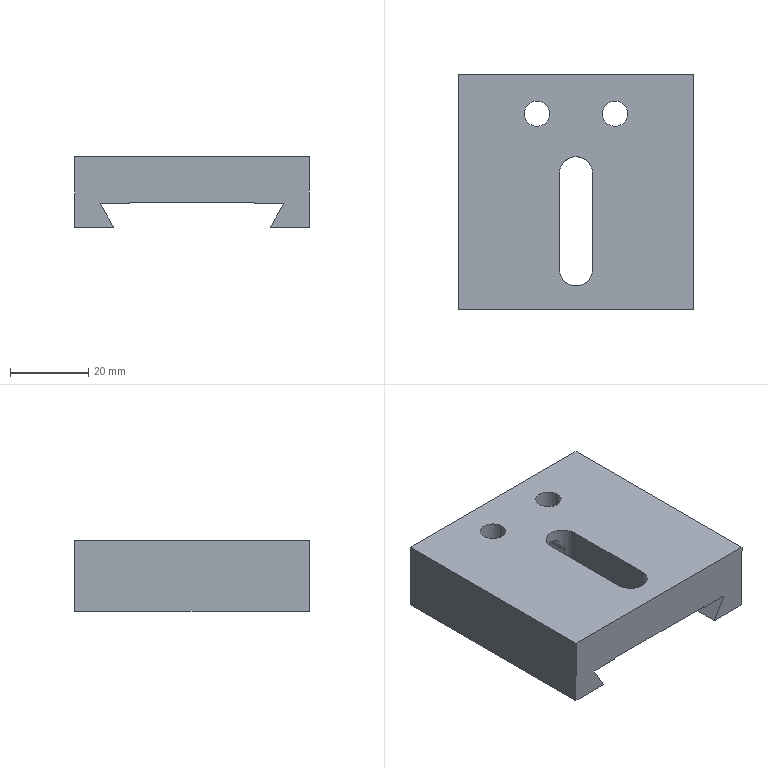Component | SolidWorks | DovetailBase2-1 | 1 solid | 30 faces | box 60 x 60 x 18 mm | volume 43120 mm3 | plane 18 | cylinder 12 | commonest cylinder face diameters 11 x4 6.5 x4 6.8 x2 8.5 x2
build123d program:
from build123d import *

# Parameters (mm, degrees)
SKETCH1_W                                          = 60
SKETCH1_H                                          = 60
BOSS_EXTRUDE1_DEPTH                                = 18
CUT_EXTRUDE1_DEPTH                                 = 72
SKETCH3_W                                          = 32
SKETCH3_H                                          = 60
CUT_EXTRUDE2_DEPTH                                 = 0.3
HOLE_SIZE_ACCORDING_TO_TYPE_1_OF_HEXAG_D           = 6.5
HOLE_SIZE_ACCORDING_TO_TYPE_1_OF_HEXAG_DEPTH       = 12.4
HOLE_SIZE_ACCORDING_TO_TYPE_1_OF_HEXAG_CBORE_D     = 11
HOLE_SIZE_ACCORDING_TO_TYPE_1_OF_HEXAG_CBORE_DEPTH = 6.5
HOLE_SIZE_ACCORDING_TO_TYPE_1_OF_HEXAG_TIP         = 1.953
CUT_EXTRUDE3_DEPTH                                 = 90.3
M8_TAPPED_HOLE1_REACH                              = 70.147
M8_TAPPED_HOLE1_BORE_R                             = 3.4


with BuildPart() as part:
    # Sketch1 → Boss-Extrude1 (new body)
    with BuildSketch(Plane.XY):
        Rectangle(SKETCH1_W, SKETCH1_H)
    extrude(amount=BOSS_EXTRUDE1_DEPTH)

    # Sketch2 → Cut-Extrude1 (cut)
    with BuildSketch(Plane(origin=(0, 30, 0), x_dir=(1, 0, 0), z_dir=(0, 1, 0))):
        Polygon((-20, -18), (-23.464, -12), (23.464, -12), (20, -18), align=None)
    extrude(amount=-CUT_EXTRUDE1_DEPTH, mode=Mode.SUBTRACT)

    # Sketch3 → Cut-Extrude2 (cut)
    with BuildSketch(Plane.XY.offset(12)):
        Rectangle(SKETCH3_W, SKETCH3_H)
    extrude(amount=-CUT_EXTRUDE2_DEPTH, mode=Mode.SUBTRACT)

    # Hole Size _according to_ Type 1 of Hexag
    with Locations(Plane(origin=(-10, 20, 11.7), x_dir=(1, 0, 0), z_dir=(0, 0, 1))):
        with Locations((0, 0), (20, 0)):
            CounterBoreHole(HOLE_SIZE_ACCORDING_TO_TYPE_1_OF_HEXAG_D / 2, HOLE_SIZE_ACCORDING_TO_TYPE_1_OF_HEXAG_CBORE_D / 2, HOLE_SIZE_ACCORDING_TO_TYPE_1_OF_HEXAG_CBORE_DEPTH, depth=HOLE_SIZE_ACCORDING_TO_TYPE_1_OF_HEXAG_DEPTH)
            with Locations((0, 0, -(HOLE_SIZE_ACCORDING_TO_TYPE_1_OF_HEXAG_DEPTH + HOLE_SIZE_ACCORDING_TO_TYPE_1_OF_HEXAG_TIP / 2))):  # 118° drill point
                Cone(0, HOLE_SIZE_ACCORDING_TO_TYPE_1_OF_HEXAG_D / 2, HOLE_SIZE_ACCORDING_TO_TYPE_1_OF_HEXAG_TIP, mode=Mode.SUBTRACT)

    # Sketch5 → Cut-Extrude3 (cut)
    with BuildSketch(Plane.XY.offset(11.7)):
        with BuildLine():
            Line((-4.25, -19.75), (-4.25, 4.75))
            ThreePointArc((-4.25, 4.75), (0, 9), (4.25, 4.75))
            Line((4.25, 4.75), (4.25, -19.75))
            ThreePointArc((4.25, -19.75), (0, -24), (-4.25, -19.75))
        make_face()
    extrude(amount=-CUT_EXTRUDE3_DEPTH, mode=Mode.SUBTRACT)

    # M8 Tapped Hole1 bore (on position points) → M8 Tapped Hole1 (cut, up to next)
    with BuildSketch(Plane(origin=(0, 30, 6), x_dir=(0, 0, 1), z_dir=(0, 1, 0)), mode=Mode.PRIVATE) as m8_tapped_hole1_sk1:
        Circle(M8_TAPPED_HOLE1_BORE_R)
    m8_tapped_hole1_tool1 = extrude(m8_tapped_hole1_sk1.sketch, amount=-M8_TAPPED_HOLE1_REACH, mode=Mode.PRIVATE) & part.part
    add(m8_tapped_hole1_tool1.solids().sort_by_distance((0, 30, 6))[0], mode=Mode.SUBTRACT)


solid = part.part

# Placed as in the assembly
solid = solid.moved(Location((-48.047, -14.04, 21), (-180, 0, 180)))
STEP:
#1=CARTESIAN_POINT('',(-1.892,-0.1984,0.7244));
#2=VERTEX_POINT('',#1);
#3=CARTESIAN_POINT('',(-1.892,-0.1984,0.4567));
#4=VERTEX_POINT('',#3);
#5=CARTESIAN_POINT('',(-1.892,-0.1984,0.7244));
#6=CARTESIAN_POINT('',(-1.882,-0.1984,0.7244));
#7=CARTESIAN_POINT('',(-1.873,-0.1992,0.7234));
#8=CARTESIAN_POINT('',(-1.855,-0.2022,0.7197));
#9=CARTESIAN_POINT('',(-1.846,-0.2044,0.7169));
#10=CARTESIAN_POINT('',(-1.83,-0.2099,0.7098));
#11=CARTESIAN_POINT('',(-1.823,-0.2131,0.7056));
#12=CARTESIAN_POINT('',(-1.808,-0.2203,0.6958));
#13=CARTESIAN_POINT('',(-1.802,-0.2243,0.6903));
#14=CARTESIAN_POINT('',(-1.79,-0.2324,0.6785));
#15=CARTESIAN_POINT('',(-1.785,-0.2366,0.672));
#16=CARTESIAN_POINT('',(-1.776,-0.2448,0.6582));
#17=CARTESIAN_POINT('',(-1.772,-0.2488,0.6509));
#18=CARTESIAN_POINT('',(-1.767,-0.2542,0.6392));
#19=CARTESIAN_POINT('',(-1.765,-0.2559,0.6352));
#20=CARTESIAN_POINT('',(-1.763,-0.259,0.6269));
#21=CARTESIAN_POINT('',(-1.762,-0.2605,0.6225));
#22=CARTESIAN_POINT('',(-1.76,-0.2628,0.6137));
#23=CARTESIAN_POINT('',(-1.759,-0.2637,0.6092));
#24=CARTESIAN_POINT('',(-1.758,-0.265,0.6));
#25=CARTESIAN_POINT('',(-1.758,-0.2653,0.5953));
#26=CARTESIAN_POINT('',(-1.758,-0.2654,0.5813));
#27=CARTESIAN_POINT('',(-1.759,-0.264,0.5721));
#28=CARTESIAN_POINT('',(-1.762,-0.2594,0.5544));
#29=CARTESIAN_POINT('',(-1.765,-0.2562,0.5461));
#30=CARTESIAN_POINT('',(-1.772,-0.2489,0.5303));
#31=CARTESIAN_POINT('',(-1.776,-0.2448,0.5229));
#32=CARTESIAN_POINT('',(-1.785,-0.2366,0.5092));
#33=CARTESIAN_POINT('',(-1.79,-0.2324,0.5027));
#34=CARTESIAN_POINT('',(-1.802,-0.2243,0.4908));
#35=CARTESIAN_POINT('',(-1.808,-0.2203,0.4853));
#36=CARTESIAN_POINT('',(-1.822,-0.2132,0.4757));
#37=CARTESIAN_POINT('',(-1.83,-0.21,0.4714));
#38=CARTESIAN_POINT('',(-1.846,-0.2045,0.4643));
#39=CARTESIAN_POINT('',(-1.855,-0.2022,0.4615));
#40=CARTESIAN_POINT('',(-1.873,-0.1992,0.4577));
#41=CARTESIAN_POINT('',(-1.882,-0.1984,0.4567));
#42=CARTESIAN_POINT('',(-1.892,-0.1984,0.4567));
#43=B_SPLINE_CURVE_WITH_KNOTS('',3,(#5,#6,#7,#8,#9,#10,#11,#12,#13,#14,#15,#16,#17,#18,#19,#20,#21,#22,#23,#24,#25,#26,#27,#28,#29,#30,#31,#32,#33,#34,#35,#36,#37,#38,#39,#40,#41,#42),.UNSPECIFIED.,.F.,.F.,(4,2,2,2,2,2,2,2,2,2,2,2,2,2,2,2,2,2,4),(0.01126,0.01196,0.01266,0.01336,0.01406,0.01477,0.01547,0.01582,0.01617,0.01652,0.01687,0.01757,0.01827,0.01897,0.01968,0.02038,0.02108,0.02178,0.02248),.UNSPECIFIED.);
#44=EDGE_CURVE('',#2,#4,#43,.T.);
#45=ORIENTED_EDGE('',*,*,#44,.F.);
#46=CARTESIAN_POINT('',(-1.892,0.6284,0.7244));
#47=VERTEX_POINT('',#46);
#48=CARTESIAN_POINT('',(-1.892,0.6284,0.7244));
#49=DIRECTION('',(-0.,1.,0.));
#50=VECTOR('',#49,39.37);
#51=LINE('',#48,#50);
#52=EDGE_CURVE('',#2,#47,#51,.T.);
#53=ORIENTED_EDGE('',*,*,#52,.T.);
#54=CARTESIAN_POINT('',(-1.892,0.6284,0.4567));
#55=VERTEX_POINT('',#54);
#56=CARTESIAN_POINT('',(-1.892,0.6284,0.5906));
#57=DIRECTION('',(-0.,1.,0.));
#58=DIRECTION('',(-0.,0.,-1.));
#59=AXIS2_PLACEMENT_3D('',#56,#57,#58);
#60=CIRCLE('',#59,0.1339);
#61=EDGE_CURVE('',#47,#55,#60,.T.);
#62=ORIENTED_EDGE('',*,*,#61,.T.);
#63=CARTESIAN_POINT('',(-1.892,0.6284,0.4567));
#64=DIRECTION('',(-0.,1.,0.));
#65=VECTOR('',#64,39.37);
#66=LINE('',#63,#65);
#67=EDGE_CURVE('',#4,#55,#66,.T.);
#68=ORIENTED_EDGE('',*,*,#67,.F.);
#69=EDGE_LOOP('',(#45,#53,#62,#68));
#70=FACE_OUTER_BOUND('',#69,.T.);
#71=CARTESIAN_POINT('',(-1.892,0.6284,0.5906));
#72=DIRECTION('',(-0.,1.,0.));
#73=DIRECTION('',(-0.,0.,-1.));
#74=AXIS2_PLACEMENT_3D('',#71,#72,#73);
#75=CYLINDRICAL_SURFACE('',#74,0.1339);
#76=ADVANCED_FACE('',(#70),#75,.F.);
#77=CARTESIAN_POINT('',(-1.281,0.2347,0.622));
#78=VERTEX_POINT('',#77);
#79=CARTESIAN_POINT('',(-1.714,0.2347,0.622));
#80=VERTEX_POINT('',#79);
#81=CARTESIAN_POINT('',(-1.498,0.2347,0.622));
#82=DIRECTION('',(-0.,0.,-1.));
#83=DIRECTION('',(-1.,0.,0.));
#84=AXIS2_PLACEMENT_3D('',#81,#82,#83);
#85=CIRCLE('',#84,0.2165);
#86=EDGE_CURVE('',#78,#80,#85,.T.);
#87=ORIENTED_EDGE('',*,*,#86,.F.);
#88=CARTESIAN_POINT('',(-1.281,0.2347,0.3661));
#89=VERTEX_POINT('',#88);
#90=CARTESIAN_POINT('',(-1.281,0.2347,0.3661));
#91=DIRECTION('',(-0.,0.,-1.));
#92=VECTOR('',#91,39.37);
#93=LINE('',#90,#92);
#94=EDGE_CURVE('',#78,#89,#93,.T.);
#95=ORIENTED_EDGE('',*,*,#94,.T.);
#96=CARTESIAN_POINT('',(-1.714,0.2347,0.3661));
#97=VERTEX_POINT('',#96);
#98=CARTESIAN_POINT('',(-1.498,0.2347,0.3661));
#99=DIRECTION('',(-0.,0.,-1.));
#100=DIRECTION('',(-1.,0.,0.));
#101=AXIS2_PLACEMENT_3D('',#98,#99,#100);
#102=CIRCLE('',#101,0.2165);
#103=EDGE_CURVE('',#89,#97,#102,.T.);
#104=ORIENTED_EDGE('',*,*,#103,.T.);
#105=CARTESIAN_POINT('',(-1.714,0.2347,0.3661));
#106=DIRECTION('',(-0.,0.,-1.));
#107=VECTOR('',#106,39.37);
#108=LINE('',#105,#107);
#109=EDGE_CURVE('',#80,#97,#108,.T.);
#110=ORIENTED_EDGE('',*,*,#109,.F.);
#111=EDGE_LOOP('',(#87,#95,#104,#110));
#112=FACE_OUTER_BOUND('',#111,.T.);
#113=CARTESIAN_POINT('',(-1.498,0.2347,0.3661));
#114=DIRECTION('',(-0.,0.,-1.));
#115=DIRECTION('',(-1.,0.,0.));
#116=AXIS2_PLACEMENT_3D('',#113,#114,#115);
#117=CYLINDRICAL_SURFACE('',#116,0.2165);
#118=ADVANCED_FACE('',(#112),#117,.F.);
#119=CARTESIAN_POINT('',(-1.626,0.2347,0.8268));
#120=VERTEX_POINT('',#119);
#121=CARTESIAN_POINT('',(-1.37,0.2347,0.8268));
#122=VERTEX_POINT('',#121);
#123=CARTESIAN_POINT('',(-1.498,0.2347,0.8268));
#124=DIRECTION('',(0.,-0.,1.));
#125=DIRECTION('',(1.,0.,-0.));
#126=AXIS2_PLACEMENT_3D('',#123,#124,#125);
#127=CIRCLE('',#126,0.128);
#128=EDGE_CURVE('',#120,#122,#127,.T.);
#129=ORIENTED_EDGE('',*,*,#128,.T.);
#130=CARTESIAN_POINT('',(-1.37,0.2347,0.622));
#131=VERTEX_POINT('',#130);
#132=CARTESIAN_POINT('',(-1.37,0.2347,0.3661));
#133=DIRECTION('',(-0.,0.,-1.));
#134=VECTOR('',#133,39.37);
#135=LINE('',#132,#134);
#136=EDGE_CURVE('',#122,#131,#135,.T.);
#137=ORIENTED_EDGE('',*,*,#136,.T.);
#138=CARTESIAN_POINT('',(-1.626,0.2347,0.622));
#139=VERTEX_POINT('',#138);
#140=CARTESIAN_POINT('',(-1.498,0.2347,0.622));
#141=DIRECTION('',(-0.,0.,-1.));
#142=DIRECTION('',(-1.,0.,0.));
#143=AXIS2_PLACEMENT_3D('',#140,#141,#142);
#144=CIRCLE('',#143,0.128);
#145=EDGE_CURVE('',#131,#139,#144,.T.);
#146=ORIENTED_EDGE('',*,*,#145,.T.);
#147=CARTESIAN_POINT('',(-1.626,0.2347,0.3661));
#148=DIRECTION('',(-0.,0.,-1.));
#149=VECTOR('',#148,39.37);
#150=LINE('',#147,#149);
#151=EDGE_CURVE('',#120,#139,#150,.T.);
#152=ORIENTED_EDGE('',*,*,#151,.F.);
#153=EDGE_LOOP('',(#129,#137,#146,#152));
#154=FACE_OUTER_BOUND('',#153,.T.);
#155=CARTESIAN_POINT('',(-1.498,0.2347,0.3661));
#156=DIRECTION('',(-0.,0.,-1.));
#157=DIRECTION('',(-1.,0.,0.));
#158=AXIS2_PLACEMENT_3D('',#155,#156,#157);
#159=CYLINDRICAL_SURFACE('',#158,0.128);
#160=ADVANCED_FACE('',(#154),#159,.F.);
#161=CARTESIAN_POINT('',(-2.069,0.2347,0.622));
#162=VERTEX_POINT('',#161);
#163=CARTESIAN_POINT('',(-2.502,0.2347,0.622));
#164=VERTEX_POINT('',#163);
#165=CARTESIAN_POINT('',(-2.285,0.2347,0.622));
#166=DIRECTION('',(-0.,0.,-1.));
#167=DIRECTION('',(-1.,0.,0.));
#168=AXIS2_PLACEMENT_3D('',#165,#166,#167);
#169=CIRCLE('',#168,0.2165);
#170=EDGE_CURVE('',#162,#164,#169,.T.);
#171=ORIENTED_EDGE('',*,*,#170,.F.);
#172=CARTESIAN_POINT('',(-2.069,0.2347,0.3661));
#173=VERTEX_POINT('',#172);
#174=CARTESIAN_POINT('',(-2.069,0.2347,0.3661));
#175=DIRECTION('',(-0.,0.,-1.));
#176=VECTOR('',#175,39.37);
#177=LINE('',#174,#176);
#178=EDGE_CURVE('',#162,#173,#177,.T.);
#179=ORIENTED_EDGE('',*,*,#178,.T.);
#180=CARTESIAN_POINT('',(-2.502,0.2347,0.3661));
#181=VERTEX_POINT('',#180);
#182=CARTESIAN_POINT('',(-2.285,0.2347,0.3661));
#183=DIRECTION('',(-0.,0.,-1.));
#184=DIRECTION('',(-1.,0.,0.));
#185=AXIS2_PLACEMENT_3D('',#182,#183,#184);
#186=CIRCLE('',#185,0.2165);
#187=EDGE_CURVE('',#173,#181,#186,.T.);
#188=ORIENTED_EDGE('',*,*,#187,.T.);
#189=CARTESIAN_POINT('',(-2.502,0.2347,0.3661));
#190=DIRECTION('',(-0.,0.,-1.));
#191=VECTOR('',#190,39.37);
#192=LINE('',#189,#191);
#193=EDGE_CURVE('',#164,#181,#192,.T.);
#194=ORIENTED_EDGE('',*,*,#193,.F.);
#195=EDGE_LOOP('',(#171,#179,#188,#194));
#196=FACE_OUTER_BOUND('',#195,.T.);
#197=CARTESIAN_POINT('',(-2.285,0.2347,0.3661));
#198=DIRECTION('',(-0.,0.,-1.));
#199=DIRECTION('',(-1.,0.,0.));
#200=AXIS2_PLACEMENT_3D('',#197,#198,#199);
#201=CYLINDRICAL_SURFACE('',#200,0.2165);
#202=ADVANCED_FACE('',(#196),#201,.F.);
#203=CARTESIAN_POINT('',(-2.413,0.2347,0.8268));
#204=VERTEX_POINT('',#203);
#205=CARTESIAN_POINT('',(-2.157,0.2347,0.8268));
#206=VERTEX_POINT('',#205);
#207=CARTESIAN_POINT('',(-2.285,0.2347,0.8268));
#208=DIRECTION('',(0.,-0.,1.));
#209=DIRECTION('',(1.,0.,-0.));
#210=AXIS2_PLACEMENT_3D('',#207,#208,#209);
#211=CIRCLE('',#210,0.128);
#212=EDGE_CURVE('',#204,#206,#211,.T.);
#213=ORIENTED_EDGE('',*,*,#212,.T.);
#214=CARTESIAN_POINT('',(-2.157,0.2347,0.622));
#215=VERTEX_POINT('',#214);
#216=CARTESIAN_POINT('',(-2.157,0.2347,0.3661));
#217=DIRECTION('',(-0.,0.,-1.));
#218=VECTOR('',#217,39.37);
#219=LINE('',#216,#218);
#220=EDGE_CURVE('',#206,#215,#219,.T.);
#221=ORIENTED_EDGE('',*,*,#220,.T.);
#222=CARTESIAN_POINT('',(-2.413,0.2347,0.622));
#223=VERTEX_POINT('',#222);
#224=CARTESIAN_POINT('',(-2.285,0.2347,0.622));
#225=DIRECTION('',(-0.,0.,-1.));
#226=DIRECTION('',(-1.,0.,0.));
#227=AXIS2_PLACEMENT_3D('',#224,#225,#226);
#228=CIRCLE('',#227,0.128);
#229=EDGE_CURVE('',#215,#223,#228,.T.);
#230=ORIENTED_EDGE('',*,*,#229,.T.);
#231=CARTESIAN_POINT('',(-2.413,0.2347,0.3661));
#232=DIRECTION('',(-0.,0.,-1.));
#233=VECTOR('',#232,39.37);
#234=LINE('',#231,#233);
#235=EDGE_CURVE('',#204,#223,#234,.T.);
#236=ORIENTED_EDGE('',*,*,#235,.F.);
#237=EDGE_LOOP('',(#213,#221,#230,#236));
#238=FACE_OUTER_BOUND('',#237,.T.);
#239=CARTESIAN_POINT('',(-2.285,0.2347,0.3661));
#240=DIRECTION('',(-0.,0.,-1.));
#241=DIRECTION('',(-1.,0.,0.));
#242=AXIS2_PLACEMENT_3D('',#239,#240,#241);
#243=CYLINDRICAL_SURFACE('',#242,0.128);
#244=ADVANCED_FACE('',(#238),#243,.F.);
#245=CARTESIAN_POINT('',(-2.815,0.6284,0.3543));
#246=VERTEX_POINT('',#245);
#247=CARTESIAN_POINT('',(-2.522,0.6284,0.3543));
#248=VERTEX_POINT('',#247);
#249=CARTESIAN_POINT('',(-0.9678,0.6284,0.3543));
#250=DIRECTION('',(1.,0.,-0.));
#251=VECTOR('',#250,39.37);
#252=LINE('',#249,#251);
#253=EDGE_CURVE('',#246,#248,#252,.T.);
#254=ORIENTED_EDGE('',*,*,#253,.T.);
#255=CARTESIAN_POINT('',(-2.522,-1.734,0.3543));
#256=VERTEX_POINT('',#255);
#257=CARTESIAN_POINT('',(-2.522,-1.734,0.3543));
#258=DIRECTION('',(-0.,1.,0.));
#259=VECTOR('',#258,39.37);
#260=LINE('',#257,#259);
#261=EDGE_CURVE('',#256,#248,#260,.T.);
#262=ORIENTED_EDGE('',*,*,#261,.F.);
#263=CARTESIAN_POINT('',(-2.815,-1.734,0.3543));
#264=VERTEX_POINT('',#263);
#265=CARTESIAN_POINT('',(-0.7105,-1.734,0.3543));
#266=DIRECTION('',(1.,0.,-0.));
#267=VECTOR('',#266,39.37);
#268=LINE('',#265,#267);
#269=EDGE_CURVE('',#264,#256,#268,.T.);
#270=ORIENTED_EDGE('',*,*,#269,.F.);
#271=CARTESIAN_POINT('',(-2.815,-2.206,0.3543));
#272=DIRECTION('',(-0.,1.,0.));
#273=VECTOR('',#272,39.37);
#274=LINE('',#271,#273);
#275=EDGE_CURVE('',#264,#246,#274,.T.);
#276=ORIENTED_EDGE('',*,*,#275,.T.);
#277=EDGE_LOOP('',(#254,#262,#270,#276));
#278=FACE_OUTER_BOUND('',#277,.T.);
#279=CARTESIAN_POINT('',(-0.9678,-2.206,0.3543));
#280=DIRECTION('',(0.,-0.,1.));
#281=DIRECTION('',(1.,0.,-0.));
#282=AXIS2_PLACEMENT_3D('',#279,#280,#281);
#283=PLANE('',#282);
#284=ADVANCED_FACE('',(#278),#283,.F.);
#285=CARTESIAN_POINT('',(-0.7105,-1.734,0.1181));
#286=VERTEX_POINT('',#285);
#287=CARTESIAN_POINT('',(-1.104,-1.734,0.1181));
#288=VERTEX_POINT('',#287);
#289=CARTESIAN_POINT('',(-0.7105,-1.734,0.1181));
#290=DIRECTION('',(-1.,-0.,0.));
#291=VECTOR('',#290,39.37);
#292=LINE('',#289,#291);
#293=EDGE_CURVE('',#286,#288,#292,.T.);
#294=ORIENTED_EDGE('',*,*,#293,.T.);
#295=CARTESIAN_POINT('',(-1.104,0.6284,0.1181));
#296=VERTEX_POINT('',#295);
#297=CARTESIAN_POINT('',(-1.104,-0.5527,0.1181));
#298=DIRECTION('',(-0.,1.,0.));
#299=VECTOR('',#298,39.37);
#300=LINE('',#297,#299);
#301=EDGE_CURVE('',#288,#296,#300,.T.);
#302=ORIENTED_EDGE('',*,*,#301,.T.);
#303=CARTESIAN_POINT('',(-0.7105,0.6284,0.1181));
#304=VERTEX_POINT('',#303);
#305=CARTESIAN_POINT('',(-0.7105,0.6284,0.1181));
#306=DIRECTION('',(1.,0.,-0.));
#307=VECTOR('',#306,39.37);
#308=LINE('',#305,#307);
#309=EDGE_CURVE('',#296,#304,#308,.T.);
#310=ORIENTED_EDGE('',*,*,#309,.T.);
#311=CARTESIAN_POINT('',(-0.7105,-1.734,0.1181));
#312=DIRECTION('',(0.,-1.,-0.));
#313=VECTOR('',#312,39.37);
#314=LINE('',#311,#313);
#315=EDGE_CURVE('',#304,#286,#314,.T.);
#316=ORIENTED_EDGE('',*,*,#315,.T.);
#317=EDGE_LOOP('',(#294,#302,#310,#316));
#318=FACE_OUTER_BOUND('',#317,.T.);
#319=CARTESIAN_POINT('',(-1.892,-0.5527,0.1181));
#320=DIRECTION('',(0.,-0.,1.));
#321=DIRECTION('',(1.,0.,-0.));
#322=AXIS2_PLACEMENT_3D('',#319,#320,#321);
#323=PLANE('',#322);
#324=ADVANCED_FACE('',(#318),#323,.F.);
#325=CARTESIAN_POINT('',(-3.073,-1.734,0.8268));
#326=VERTEX_POINT('',#325);
#327=CARTESIAN_POINT('',(-3.073,0.6284,0.8268));
#328=VERTEX_POINT('',#327);
#329=CARTESIAN_POINT('',(-3.073,-1.734,0.8268));
#330=DIRECTION('',(-0.,1.,0.));
#331=VECTOR('',#330,39.37);
#332=LINE('',#329,#331);
#333=EDGE_CURVE('',#326,#328,#332,.T.);
#334=ORIENTED_EDGE('',*,*,#333,.T.);
#335=CARTESIAN_POINT('',(-3.073,0.6284,0.1181));
#336=VERTEX_POINT('',#335);
#337=CARTESIAN_POINT('',(-3.073,0.6284,0.1181));
#338=DIRECTION('',(0.,-0.,1.));
#339=VECTOR('',#338,39.37);
#340=LINE('',#337,#339);
#341=EDGE_CURVE('',#336,#328,#340,.T.);
#342=ORIENTED_EDGE('',*,*,#341,.F.);
#343=CARTESIAN_POINT('',(-3.073,-1.734,0.1181));
#344=VERTEX_POINT('',#343);
#345=CARTESIAN_POINT('',(-3.073,-1.734,0.1181));
#346=DIRECTION('',(-0.,1.,0.));
#347=VECTOR('',#346,39.37);
#348=LINE('',#345,#347);
#349=EDGE_CURVE('',#344,#336,#348,.T.);
#350=ORIENTED_EDGE('',*,*,#349,.F.);
#351=CARTESIAN_POINT('',(-3.073,-1.734,0.1181));
#352=DIRECTION('',(0.,-0.,1.));
#353=VECTOR('',#352,39.37);
#354=LINE('',#351,#353);
#355=EDGE_CURVE('',#344,#326,#354,.T.);
#356=ORIENTED_EDGE('',*,*,#355,.T.);
#357=EDGE_LOOP('',(#334,#342,#350,#356));
#358=FACE_OUTER_BOUND('',#357,.T.);
#359=CARTESIAN_POINT('',(-3.073,-1.734,0.1181));
#360=DIRECTION('',(1.,0.,-0.));
#361=DIRECTION('',(-0.,0.,-1.));
#362=AXIS2_PLACEMENT_3D('',#359,#360,#361);
#363=PLANE('',#362);
#364=ADVANCED_FACE('',(#358),#363,.F.);
#365=CARTESIAN_POINT('',(-1.892,0.6284,0.5906));
#366=DIRECTION('',(-0.,1.,0.));
#367=DIRECTION('',(-0.,0.,-1.));
#368=AXIS2_PLACEMENT_3D('',#365,#366,#367);
#369=CIRCLE('',#368,0.1339);
#370=EDGE_CURVE('',#55,#47,#369,.T.);
#371=ORIENTED_EDGE('',*,*,#370,.F.);
#372=ORIENTED_EDGE('',*,*,#61,.F.);
#373=EDGE_LOOP('',(#371,#372));
#374=FACE_BOUND('',#373,.T.);
#375=CARTESIAN_POINT('',(-2.522,0.6284,0.3661));
#376=VERTEX_POINT('',#375);
#377=CARTESIAN_POINT('',(-1.262,0.6284,0.3661));
#378=VERTEX_POINT('',#377);
#379=CARTESIAN_POINT('',(-1.262,0.6284,0.3661));
#380=DIRECTION('',(1.,0.,-0.));
#381=VECTOR('',#380,39.37);
#382=LINE('',#379,#381);
#383=EDGE_CURVE('',#376,#378,#382,.T.);
#384=ORIENTED_EDGE('',*,*,#383,.F.);
#385=CARTESIAN_POINT('',(-2.522,0.6284,0.3661));
#386=DIRECTION('',(-0.,0.,-1.));
#387=VECTOR('',#386,39.37);
#388=LINE('',#385,#387);
#389=EDGE_CURVE('',#376,#248,#388,.T.);
#390=ORIENTED_EDGE('',*,*,#389,.T.);
#391=ORIENTED_EDGE('',*,*,#253,.F.);
#392=CARTESIAN_POINT('',(-2.679,0.6284,0.1181));
#393=VERTEX_POINT('',#392);
#394=CARTESIAN_POINT('',(-2.815,0.6284,0.3543));
#395=DIRECTION('',(-0.5,-0.,0.866));
#396=VECTOR('',#395,39.37);
#397=LINE('',#394,#396);
#398=EDGE_CURVE('',#393,#246,#397,.T.);
#399=ORIENTED_EDGE('',*,*,#398,.F.);
#400=CARTESIAN_POINT('',(-0.7105,0.6284,0.1181));
#401=DIRECTION('',(1.,0.,-0.));
#402=VECTOR('',#401,39.37);
#403=LINE('',#400,#402);
#404=EDGE_CURVE('',#336,#393,#403,.T.);
#405=ORIENTED_EDGE('',*,*,#404,.F.);
#406=ORIENTED_EDGE('',*,*,#341,.T.);
#407=CARTESIAN_POINT('',(-0.7105,0.6284,0.8268));
#408=VERTEX_POINT('',#407);
#409=CARTESIAN_POINT('',(-0.7105,0.6284,0.8268));
#410=DIRECTION('',(1.,0.,-0.));
#411=VECTOR('',#410,39.37);
#412=LINE('',#409,#411);
#413=EDGE_CURVE('',#328,#408,#412,.T.);
#414=ORIENTED_EDGE('',*,*,#413,.T.);
#415=CARTESIAN_POINT('',(-0.7105,0.6284,0.1181));
#416=DIRECTION('',(0.,-0.,1.));
#417=VECTOR('',#416,39.37);
#418=LINE('',#415,#417);
#419=EDGE_CURVE('',#304,#408,#418,.T.);
#420=ORIENTED_EDGE('',*,*,#419,.F.);
#421=ORIENTED_EDGE('',*,*,#309,.F.);
#422=CARTESIAN_POINT('',(-0.9678,0.6284,0.3543));
#423=VERTEX_POINT('',#422);
#424=CARTESIAN_POINT('',(-1.104,0.6284,0.1181));
#425=DIRECTION('',(-0.5,-0.,-0.866));
#426=VECTOR('',#425,39.37);
#427=LINE('',#424,#426);
#428=EDGE_CURVE('',#423,#296,#427,.T.);
#429=ORIENTED_EDGE('',*,*,#428,.F.);
#430=CARTESIAN_POINT('',(-1.262,0.6284,0.3543));
#431=VERTEX_POINT('',#430);
#432=CARTESIAN_POINT('',(-0.9678,0.6284,0.3543));
#433=DIRECTION('',(1.,0.,-0.));
#434=VECTOR('',#433,39.37);
#435=LINE('',#432,#434);
#436=EDGE_CURVE('',#431,#423,#435,.T.);
#437=ORIENTED_EDGE('',*,*,#436,.F.);
#438=CARTESIAN_POINT('',(-1.262,0.6284,0.3661));
#439=DIRECTION('',(-0.,0.,-1.));
#440=VECTOR('',#439,39.37);
#441=LINE('',#438,#440);
#442=EDGE_CURVE('',#378,#431,#441,.T.);
#443=ORIENTED_EDGE('',*,*,#442,.F.);
#444=EDGE_LOOP('',(#384,#390,#391,#399,#405,#406,#414,#420,#421,#429,#437,#443));
#445=FACE_OUTER_BOUND('',#444,.T.);
#446=CARTESIAN_POINT('',(-0.7105,0.6284,0.1181));
#447=DIRECTION('',(0.,-1.,-0.));
#448=DIRECTION('',(0.,-0.,1.));
#449=AXIS2_PLACEMENT_3D('',#446,#447,#448);
#450=PLANE('',#449);
#451=ADVANCED_FACE('',(#374,#445),#450,.F.);
#452=CARTESIAN_POINT('',(-0.7105,-1.734,0.8268));
#453=VERTEX_POINT('',#452);
#454=CARTESIAN_POINT('',(-0.7105,-1.734,0.8268));
#455=DIRECTION('',(0.,-1.,-0.));
#456=VECTOR('',#455,39.37);
#457=LINE('',#454,#456);
#458=EDGE_CURVE('',#408,#453,#457,.T.);
#459=ORIENTED_EDGE('',*,*,#458,.T.);
#460=CARTESIAN_POINT('',(-0.7105,-1.734,0.1181));
#461=DIRECTION('',(0.,-0.,1.));
#462=VECTOR('',#461,39.37);
#463=LINE('',#460,#462);
#464=EDGE_CURVE('',#286,#453,#463,.T.);
#465=ORIENTED_EDGE('',*,*,#464,.F.);
#466=ORIENTED_EDGE('',*,*,#315,.F.);
#467=ORIENTED_EDGE('',*,*,#419,.T.);
#468=EDGE_LOOP('',(#459,#465,#466,#467));
#469=FACE_OUTER_BOUND('',#468,.T.);
#470=CARTESIAN_POINT('',(-0.7105,-1.734,0.1181));
#471=DIRECTION('',(-1.,-0.,0.));
#472=DIRECTION('',(0.,-0.,1.));
#473=AXIS2_PLACEMENT_3D('',#470,#471,#472);
#474=PLANE('',#473);
#475=ADVANCED_FACE('',(#469),#474,.F.);
#476=ORIENTED_EDGE('',*,*,#269,.T.);
#477=CARTESIAN_POINT('',(-2.522,-1.734,0.3661));
#478=VERTEX_POINT('',#477);
#479=CARTESIAN_POINT('',(-2.522,-1.734,0.3661));
#480=DIRECTION('',(-0.,0.,-1.));
#481=VECTOR('',#480,39.37);
#482=LINE('',#479,#481);
#483=EDGE_CURVE('',#478,#256,#482,.T.);
#484=ORIENTED_EDGE('',*,*,#483,.F.);
#485=CARTESIAN_POINT('',(-1.262,-1.734,0.3661));
#486=VERTEX_POINT('',#485);
#487=CARTESIAN_POINT('',(-1.262,-1.734,0.3661));
#488=DIRECTION('',(-1.,-0.,0.));
#489=VECTOR('',#488,39.37);
#490=LINE('',#487,#489);
#491=EDGE_CURVE('',#486,#478,#490,.T.);
#492=ORIENTED_EDGE('',*,*,#491,.F.);
#493=CARTESIAN_POINT('',(-1.262,-1.734,0.3543));
#494=VERTEX_POINT('',#493);
#495=CARTESIAN_POINT('',(-1.262,-1.734,0.3661));
#496=DIRECTION('',(-0.,0.,-1.));
#497=VECTOR('',#496,39.37);
#498=LINE('',#495,#497);
#499=EDGE_CURVE('',#486,#494,#498,.T.);
#500=ORIENTED_EDGE('',*,*,#499,.T.);
#501=CARTESIAN_POINT('',(-0.9678,-1.734,0.3543));
#502=VERTEX_POINT('',#501);
#503=CARTESIAN_POINT('',(-0.7105,-1.734,0.3543));
#504=DIRECTION('',(1.,0.,-0.));
#505=VECTOR('',#504,39.37);
#506=LINE('',#503,#505);
#507=EDGE_CURVE('',#494,#502,#506,.T.);
#508=ORIENTED_EDGE('',*,*,#507,.T.);
#509=CARTESIAN_POINT('',(-1.006,-1.734,0.2886));
#510=DIRECTION('',(-0.5,-0.,-0.866));
#511=VECTOR('',#510,39.37);
#512=LINE('',#509,#511);
#513=EDGE_CURVE('',#502,#288,#512,.T.);
#514=ORIENTED_EDGE('',*,*,#513,.T.);
#515=ORIENTED_EDGE('',*,*,#293,.F.);
#516=ORIENTED_EDGE('',*,*,#464,.T.);
#517=CARTESIAN_POINT('',(-0.7105,-1.734,0.8268));
#518=DIRECTION('',(-1.,-0.,0.));
#519=VECTOR('',#518,39.37);
#520=LINE('',#517,#519);
#521=EDGE_CURVE('',#453,#326,#520,.T.);
#522=ORIENTED_EDGE('',*,*,#521,.T.);
#523=ORIENTED_EDGE('',*,*,#355,.F.);
#524=CARTESIAN_POINT('',(-2.679,-1.734,0.1181));
#525=VERTEX_POINT('',#524);
#526=CARTESIAN_POINT('',(-0.7105,-1.734,0.1181));
#527=DIRECTION('',(-1.,-0.,0.));
#528=VECTOR('',#527,39.37);
#529=LINE('',#526,#528);
#530=EDGE_CURVE('',#525,#344,#529,.T.);
#531=ORIENTED_EDGE('',*,*,#530,.F.);
#532=CARTESIAN_POINT('',(-2.187,-1.734,-0.7343));
#533=DIRECTION('',(-0.5,-0.,0.866));
#534=VECTOR('',#533,39.37);
#535=LINE('',#532,#534);
#536=EDGE_CURVE('',#525,#264,#535,.T.);
#537=ORIENTED_EDGE('',*,*,#536,.T.);
#538=EDGE_LOOP('',(#476,#484,#492,#500,#508,#514,#515,#516,#522,#523,#531,#537));
#539=FACE_OUTER_BOUND('',#538,.T.);
#540=CARTESIAN_POINT('',(-0.7105,-1.734,0.1181));
#541=DIRECTION('',(-0.,1.,0.));
#542=DIRECTION('',(-0.,0.,-1.));
#543=AXIS2_PLACEMENT_3D('',#540,#541,#542);
#544=PLANE('',#543);
#545=ADVANCED_FACE('',(#539),#544,.F.);
#546=ORIENTED_EDGE('',*,*,#404,.T.);
#547=CARTESIAN_POINT('',(-2.679,-0.5527,0.1181));
#548=DIRECTION('',(0.,-1.,-0.));
#549=VECTOR('',#548,39.37);
#550=LINE('',#547,#549);
#551=EDGE_CURVE('',#393,#525,#550,.T.);
#552=ORIENTED_EDGE('',*,*,#551,.T.);
#553=ORIENTED_EDGE('',*,*,#530,.T.);
#554=ORIENTED_EDGE('',*,*,#349,.T.);
#555=EDGE_LOOP('',(#546,#552,#553,#554));
#556=FACE_OUTER_BOUND('',#555,.T.);
#557=CARTESIAN_POINT('',(-1.892,-0.5527,0.1181));
#558=DIRECTION('',(0.,-0.,1.));
#559=DIRECTION('',(1.,0.,-0.));
#560=AXIS2_PLACEMENT_3D('',#557,#558,#559);
#561=PLANE('',#560);
#562=ADVANCED_FACE('',(#556),#561,.F.);
#563=CARTESIAN_POINT('',(-2.059,-1.33,0.8268));
#564=VERTEX_POINT('',#563);
#565=CARTESIAN_POINT('',(-1.724,-1.33,0.8268));
#566=VERTEX_POINT('',#565);
#567=CARTESIAN_POINT('',(-1.892,-1.33,0.8268));
#568=DIRECTION('',(0.,-0.,1.));
#569=DIRECTION('',(1.,0.,-0.));
#570=AXIS2_PLACEMENT_3D('',#567,#568,#569);
#571=CIRCLE('',#570,0.1673);
#572=EDGE_CURVE('',#564,#566,#571,.T.);
#573=ORIENTED_EDGE('',*,*,#572,.F.);
#574=CARTESIAN_POINT('',(-2.059,-0.3657,0.8268));
#575=VERTEX_POINT('',#574);
#576=CARTESIAN_POINT('',(-2.059,-0.5527,0.8268));
#577=DIRECTION('',(0.,-1.,-0.));
#578=VECTOR('',#577,39.37);
#579=LINE('',#576,#578);
#580=EDGE_CURVE('',#575,#564,#579,.T.);
#581=ORIENTED_EDGE('',*,*,#580,.F.);
#582=CARTESIAN_POINT('',(-1.724,-0.3657,0.8268));
#583=VERTEX_POINT('',#582);
#584=CARTESIAN_POINT('',(-1.892,-0.3657,0.8268));
#585=DIRECTION('',(0.,-0.,1.));
#586=DIRECTION('',(1.,0.,-0.));
#587=AXIS2_PLACEMENT_3D('',#584,#585,#586);
#588=CIRCLE('',#587,0.1673);
#589=EDGE_CURVE('',#583,#575,#588,.T.);
#590=ORIENTED_EDGE('',*,*,#589,.F.);
#591=CARTESIAN_POINT('',(-1.724,-0.5527,0.8268));
#592=DIRECTION('',(-0.,1.,0.));
#593=VECTOR('',#592,39.37);
#594=LINE('',#591,#593);
#595=EDGE_CURVE('',#566,#583,#594,.T.);
#596=ORIENTED_EDGE('',*,*,#595,.F.);
#597=EDGE_LOOP('',(#573,#581,#590,#596));
#598=FACE_BOUND('',#597,.T.);
#599=ORIENTED_EDGE('',*,*,#128,.F.);
#600=CARTESIAN_POINT('',(-1.498,0.2347,0.8268));
#601=DIRECTION('',(0.,-0.,1.));
#602=DIRECTION('',(1.,0.,-0.));
#603=AXIS2_PLACEMENT_3D('',#600,#601,#602);
#604=CIRCLE('',#603,0.128);
#605=EDGE_CURVE('',#122,#120,#604,.T.);
#606=ORIENTED_EDGE('',*,*,#605,.F.);
#607=EDGE_LOOP('',(#599,#606));
#608=FACE_BOUND('',#607,.T.);
#609=ORIENTED_EDGE('',*,*,#212,.F.);
#610=CARTESIAN_POINT('',(-2.285,0.2347,0.8268));
#611=DIRECTION('',(0.,-0.,1.));
#612=DIRECTION('',(1.,0.,-0.));
#613=AXIS2_PLACEMENT_3D('',#610,#611,#612);
#614=CIRCLE('',#613,0.128);
#615=EDGE_CURVE('',#206,#204,#614,.T.);
#616=ORIENTED_EDGE('',*,*,#615,.F.);
#617=EDGE_LOOP('',(#609,#616));
#618=FACE_BOUND('',#617,.T.);
#619=ORIENTED_EDGE('',*,*,#333,.F.);
#620=ORIENTED_EDGE('',*,*,#521,.F.);
#621=ORIENTED_EDGE('',*,*,#458,.F.);
#622=ORIENTED_EDGE('',*,*,#413,.F.);
#623=EDGE_LOOP('',(#619,#620,#621,#622));
#624=FACE_OUTER_BOUND('',#623,.T.);
#625=CARTESIAN_POINT('',(-1.892,-0.5527,0.8268));
#626=DIRECTION('',(0.,-0.,1.));
#627=DIRECTION('',(1.,0.,-0.));
#628=AXIS2_PLACEMENT_3D('',#625,#626,#627);
#629=PLANE('',#628);
#630=ADVANCED_FACE('',(#598,#608,#618,#624),#629,.T.);
#631=ORIENTED_EDGE('',*,*,#507,.F.);
#632=CARTESIAN_POINT('',(-1.262,-1.734,0.3543));
#633=DIRECTION('',(0.,-1.,-0.));
#634=VECTOR('',#633,39.37);
#635=LINE('',#632,#634);
#636=EDGE_CURVE('',#431,#494,#635,.T.);
#637=ORIENTED_EDGE('',*,*,#636,.F.);
#638=ORIENTED_EDGE('',*,*,#436,.T.);
#639=CARTESIAN_POINT('',(-0.9678,-2.206,0.3543));
#640=DIRECTION('',(-0.,1.,0.));
#641=VECTOR('',#640,39.37);
#642=LINE('',#639,#641);
#643=EDGE_CURVE('',#502,#423,#642,.T.);
#644=ORIENTED_EDGE('',*,*,#643,.F.);
#645=EDGE_LOOP('',(#631,#637,#638,#644));
#646=FACE_OUTER_BOUND('',#645,.T.);
#647=CARTESIAN_POINT('',(-0.9678,-2.206,0.3543));
#648=DIRECTION('',(0.,-0.,1.));
#649=DIRECTION('',(1.,0.,-0.));
#650=AXIS2_PLACEMENT_3D('',#647,#648,#649);
#651=PLANE('',#650);
#652=ADVANCED_FACE('',(#646),#651,.F.);
#653=ORIENTED_EDGE('',*,*,#643,.T.);
#654=ORIENTED_EDGE('',*,*,#428,.T.);
#655=ORIENTED_EDGE('',*,*,#301,.F.);
#656=ORIENTED_EDGE('',*,*,#513,.F.);
#657=EDGE_LOOP('',(#653,#654,#655,#656));
#658=FACE_OUTER_BOUND('',#657,.T.);
#659=CARTESIAN_POINT('',(-1.104,-2.206,0.1181));
#660=DIRECTION('',(0.866,0.,-0.5));
#661=DIRECTION('',(-0.5,-0.,-0.866));
#662=AXIS2_PLACEMENT_3D('',#659,#660,#661);
#663=PLANE('',#662);
#664=ADVANCED_FACE('',(#658),#663,.F.);
#665=ORIENTED_EDGE('',*,*,#551,.F.);
#666=ORIENTED_EDGE('',*,*,#398,.T.);
#667=ORIENTED_EDGE('',*,*,#275,.F.);
#668=ORIENTED_EDGE('',*,*,#536,.F.);
#669=EDGE_LOOP('',(#665,#666,#667,#668));
#670=FACE_OUTER_BOUND('',#669,.T.);
#671=CARTESIAN_POINT('',(-2.815,-2.206,0.3543));
#672=DIRECTION('',(-0.866,-0.,-0.5));
#673=DIRECTION('',(-0.5,-0.,0.866));
#674=AXIS2_PLACEMENT_3D('',#671,#672,#673);
#675=PLANE('',#674);
#676=ADVANCED_FACE('',(#670),#675,.F.);
#677=ORIENTED_EDGE('',*,*,#261,.T.);
#678=ORIENTED_EDGE('',*,*,#389,.F.);
#679=CARTESIAN_POINT('',(-2.522,-1.734,0.3661));
#680=DIRECTION('',(-0.,1.,0.));
#681=VECTOR('',#680,39.37);
#682=LINE('',#679,#681);
#683=EDGE_CURVE('',#478,#376,#682,.T.);
#684=ORIENTED_EDGE('',*,*,#683,.F.);
#685=ORIENTED_EDGE('',*,*,#483,.T.);
#686=EDGE_LOOP('',(#677,#678,#684,#685));
#687=FACE_OUTER_BOUND('',#686,.T.);
#688=CARTESIAN_POINT('',(-2.522,-1.734,0.3661));
#689=DIRECTION('',(-1.,-0.,0.));
#690=DIRECTION('',(0.,-0.,1.));
#691=AXIS2_PLACEMENT_3D('',#688,#689,#690);
#692=PLANE('',#691);
#693=ADVANCED_FACE('',(#687),#692,.F.);
#694=ORIENTED_EDGE('',*,*,#636,.T.);
#695=ORIENTED_EDGE('',*,*,#499,.F.);
#696=CARTESIAN_POINT('',(-1.262,-1.734,0.3661));
#697=DIRECTION('',(0.,-1.,-0.));
#698=VECTOR('',#697,39.37);
#699=LINE('',#696,#698);
#700=EDGE_CURVE('',#378,#486,#699,.T.);
#701=ORIENTED_EDGE('',*,*,#700,.F.);
#702=ORIENTED_EDGE('',*,*,#442,.T.);
#703=EDGE_LOOP('',(#694,#695,#701,#702));
#704=FACE_OUTER_BOUND('',#703,.T.);
#705=CARTESIAN_POINT('',(-1.262,-1.734,0.3661));
#706=DIRECTION('',(1.,0.,-0.));
#707=DIRECTION('',(-0.,0.,-1.));
#708=AXIS2_PLACEMENT_3D('',#705,#706,#707);
#709=PLANE('',#708);
#710=ADVANCED_FACE('',(#704),#709,.F.);
#711=CARTESIAN_POINT('',(-2.059,-1.33,0.3661));
#712=VERTEX_POINT('',#711);
#713=CARTESIAN_POINT('',(-2.059,-0.3657,0.3661));
#714=VERTEX_POINT('',#713);
#715=CARTESIAN_POINT('',(-2.059,-1.33,0.3661));
#716=DIRECTION('',(-0.,1.,0.));
#717=VECTOR('',#716,39.37);
#718=LINE('',#715,#717);
#719=EDGE_CURVE('',#712,#714,#718,.T.);
#720=ORIENTED_EDGE('',*,*,#719,.F.);
#721=CARTESIAN_POINT('',(-1.724,-1.33,0.3661));
#722=VERTEX_POINT('',#721);
#723=CARTESIAN_POINT('',(-1.892,-1.33,0.3661));
#724=DIRECTION('',(-0.,0.,-1.));
#725=DIRECTION('',(-1.,0.,0.));
#726=AXIS2_PLACEMENT_3D('',#723,#724,#725);
#727=CIRCLE('',#726,0.1673);
#728=EDGE_CURVE('',#722,#712,#727,.T.);
#729=ORIENTED_EDGE('',*,*,#728,.F.);
#730=CARTESIAN_POINT('',(-1.724,-0.3657,0.3661));
#731=VERTEX_POINT('',#730);
#732=CARTESIAN_POINT('',(-1.724,-1.33,0.3661));
#733=DIRECTION('',(0.,-1.,-0.));
#734=VECTOR('',#733,39.37);
#735=LINE('',#732,#734);
#736=EDGE_CURVE('',#731,#722,#735,.T.);
#737=ORIENTED_EDGE('',*,*,#736,.F.);
#738=CARTESIAN_POINT('',(-1.892,-0.3657,0.3661));
#739=DIRECTION('',(-0.,0.,-1.));
#740=DIRECTION('',(-1.,0.,0.));
#741=AXIS2_PLACEMENT_3D('',#738,#739,#740);
#742=CIRCLE('',#741,0.1673);
#743=EDGE_CURVE('',#714,#731,#742,.T.);
#744=ORIENTED_EDGE('',*,*,#743,.F.);
#745=EDGE_LOOP('',(#720,#729,#737,#744));
#746=FACE_BOUND('',#745,.T.);
#747=CARTESIAN_POINT('',(-1.498,0.2347,0.3661));
#748=DIRECTION('',(-0.,0.,-1.));
#749=DIRECTION('',(-1.,0.,0.));
#750=AXIS2_PLACEMENT_3D('',#747,#748,#749);
#751=CIRCLE('',#750,0.2165);
#752=EDGE_CURVE('',#97,#89,#751,.T.);
#753=ORIENTED_EDGE('',*,*,#752,.F.);
#754=ORIENTED_EDGE('',*,*,#103,.F.);
#755=EDGE_LOOP('',(#753,#754));
#756=FACE_BOUND('',#755,.T.);
#757=CARTESIAN_POINT('',(-2.285,0.2347,0.3661));
#758=DIRECTION('',(-0.,0.,-1.));
#759=DIRECTION('',(-1.,0.,0.));
#760=AXIS2_PLACEMENT_3D('',#757,#758,#759);
#761=CIRCLE('',#760,0.2165);
#762=EDGE_CURVE('',#181,#173,#761,.T.);
#763=ORIENTED_EDGE('',*,*,#762,.F.);
#764=ORIENTED_EDGE('',*,*,#187,.F.);
#765=EDGE_LOOP('',(#763,#764));
#766=FACE_BOUND('',#765,.T.);
#767=ORIENTED_EDGE('',*,*,#683,.T.);
#768=ORIENTED_EDGE('',*,*,#383,.T.);
#769=ORIENTED_EDGE('',*,*,#700,.T.);
#770=ORIENTED_EDGE('',*,*,#491,.T.);
#771=EDGE_LOOP('',(#767,#768,#769,#770));
#772=FACE_OUTER_BOUND('',#771,.T.);
#773=CARTESIAN_POINT('',(-1.892,-0.5527,0.3661));
#774=DIRECTION('',(0.,-0.,1.));
#775=DIRECTION('',(1.,0.,-0.));
#776=AXIS2_PLACEMENT_3D('',#773,#774,#775);
#777=PLANE('',#776);
#778=ADVANCED_FACE('',(#746,#756,#766,#772),#777,.F.);
#779=ORIENTED_EDGE('',*,*,#220,.F.);
#780=ORIENTED_EDGE('',*,*,#615,.T.);
#781=ORIENTED_EDGE('',*,*,#235,.T.);
#782=CARTESIAN_POINT('',(-2.285,0.2347,0.622));
#783=DIRECTION('',(-0.,0.,-1.));
#784=DIRECTION('',(-1.,0.,0.));
#785=AXIS2_PLACEMENT_3D('',#782,#783,#784);
#786=CIRCLE('',#785,0.128);
#787=EDGE_CURVE('',#223,#215,#786,.T.);
#788=ORIENTED_EDGE('',*,*,#787,.T.);
#789=EDGE_LOOP('',(#779,#780,#781,#788));
#790=FACE_OUTER_BOUND('',#789,.T.);
#791=CARTESIAN_POINT('',(-2.285,0.2347,0.3661));
#792=DIRECTION('',(-0.,0.,-1.));
#793=DIRECTION('',(-1.,0.,0.));
#794=AXIS2_PLACEMENT_3D('',#791,#792,#793);
#795=CYLINDRICAL_SURFACE('',#794,0.128);
#796=ADVANCED_FACE('',(#790),#795,.F.);
#797=ORIENTED_EDGE('',*,*,#787,.F.);
#798=ORIENTED_EDGE('',*,*,#229,.F.);
#799=EDGE_LOOP('',(#797,#798));
#800=FACE_BOUND('',#799,.T.);
#801=CARTESIAN_POINT('',(-2.285,0.2347,0.622));
#802=DIRECTION('',(-0.,0.,-1.));
#803=DIRECTION('',(-1.,0.,0.));
#804=AXIS2_PLACEMENT_3D('',#801,#802,#803);
#805=CIRCLE('',#804,0.2165);
#806=EDGE_CURVE('',#164,#162,#805,.T.);
#807=ORIENTED_EDGE('',*,*,#806,.T.);
#808=ORIENTED_EDGE('',*,*,#170,.T.);
#809=EDGE_LOOP('',(#807,#808));
#810=FACE_OUTER_BOUND('',#809,.T.);
#811=CARTESIAN_POINT('',(-2.413,0.2347,0.622));
#812=DIRECTION('',(0.,-0.,1.));
#813=DIRECTION('',(1.,0.,-0.));
#814=AXIS2_PLACEMENT_3D('',#811,#812,#813);
#815=PLANE('',#814);
#816=ADVANCED_FACE('',(#800,#810),#815,.F.);
#817=ORIENTED_EDGE('',*,*,#178,.F.);
#818=ORIENTED_EDGE('',*,*,#806,.F.);
#819=ORIENTED_EDGE('',*,*,#193,.T.);
#820=ORIENTED_EDGE('',*,*,#762,.T.);
#821=EDGE_LOOP('',(#817,#818,#819,#820));
#822=FACE_OUTER_BOUND('',#821,.T.);
#823=CARTESIAN_POINT('',(-2.285,0.2347,0.3661));
#824=DIRECTION('',(-0.,0.,-1.));
#825=DIRECTION('',(-1.,0.,0.));
#826=AXIS2_PLACEMENT_3D('',#823,#824,#825);
#827=CYLINDRICAL_SURFACE('',#826,0.2165);
#828=ADVANCED_FACE('',(#822),#827,.F.);
#829=ORIENTED_EDGE('',*,*,#136,.F.);
#830=ORIENTED_EDGE('',*,*,#605,.T.);
#831=ORIENTED_EDGE('',*,*,#151,.T.);
#832=CARTESIAN_POINT('',(-1.498,0.2347,0.622));
#833=DIRECTION('',(-0.,0.,-1.));
#834=DIRECTION('',(-1.,0.,0.));
#835=AXIS2_PLACEMENT_3D('',#832,#833,#834);
#836=CIRCLE('',#835,0.128);
#837=EDGE_CURVE('',#139,#131,#836,.T.);
#838=ORIENTED_EDGE('',*,*,#837,.T.);
#839=EDGE_LOOP('',(#829,#830,#831,#838));
#840=FACE_OUTER_BOUND('',#839,.T.);
#841=CARTESIAN_POINT('',(-1.498,0.2347,0.3661));
#842=DIRECTION('',(-0.,0.,-1.));
#843=DIRECTION('',(-1.,0.,0.));
#844=AXIS2_PLACEMENT_3D('',#841,#842,#843);
#845=CYLINDRICAL_SURFACE('',#844,0.128);
#846=ADVANCED_FACE('',(#840),#845,.F.);
#847=ORIENTED_EDGE('',*,*,#837,.F.);
#848=ORIENTED_EDGE('',*,*,#145,.F.);
#849=EDGE_LOOP('',(#847,#848));
#850=FACE_BOUND('',#849,.T.);
#851=CARTESIAN_POINT('',(-1.498,0.2347,0.622));
#852=DIRECTION('',(-0.,0.,-1.));
#853=DIRECTION('',(-1.,0.,0.));
#854=AXIS2_PLACEMENT_3D('',#851,#852,#853);
#855=CIRCLE('',#854,0.2165);
#856=EDGE_CURVE('',#80,#78,#855,.T.);
#857=ORIENTED_EDGE('',*,*,#856,.T.);
#858=ORIENTED_EDGE('',*,*,#86,.T.);
#859=EDGE_LOOP('',(#857,#858));
#860=FACE_OUTER_BOUND('',#859,.T.);
#861=CARTESIAN_POINT('',(-1.626,0.2347,0.622));
#862=DIRECTION('',(0.,-0.,1.));
#863=DIRECTION('',(1.,0.,-0.));
#864=AXIS2_PLACEMENT_3D('',#861,#862,#863);
#865=PLANE('',#864);
#866=ADVANCED_FACE('',(#850,#860),#865,.F.);
#867=ORIENTED_EDGE('',*,*,#94,.F.);
#868=ORIENTED_EDGE('',*,*,#856,.F.);
#869=ORIENTED_EDGE('',*,*,#109,.T.);
#870=ORIENTED_EDGE('',*,*,#752,.T.);
#871=EDGE_LOOP('',(#867,#868,#869,#870));
#872=FACE_OUTER_BOUND('',#871,.T.);
#873=CARTESIAN_POINT('',(-1.498,0.2347,0.3661));
#874=DIRECTION('',(-0.,0.,-1.));
#875=DIRECTION('',(-1.,0.,0.));
#876=AXIS2_PLACEMENT_3D('',#873,#874,#875);
#877=CYLINDRICAL_SURFACE('',#876,0.2165);
#878=ADVANCED_FACE('',(#872),#877,.F.);
#879=ORIENTED_EDGE('',*,*,#572,.T.);
#880=CARTESIAN_POINT('',(-1.724,-1.33,3.921));
#881=DIRECTION('',(-0.,0.,-1.));
#882=VECTOR('',#881,39.37);
#883=LINE('',#880,#882);
#884=EDGE_CURVE('',#566,#722,#883,.T.);
#885=ORIENTED_EDGE('',*,*,#884,.T.);
#886=ORIENTED_EDGE('',*,*,#728,.T.);
#887=CARTESIAN_POINT('',(-2.059,-1.33,3.921));
#888=DIRECTION('',(-0.,0.,-1.));
#889=VECTOR('',#888,39.37);
#890=LINE('',#887,#889);
#891=EDGE_CURVE('',#564,#712,#890,.T.);
#892=ORIENTED_EDGE('',*,*,#891,.F.);
#893=EDGE_LOOP('',(#879,#885,#886,#892));
#894=FACE_OUTER_BOUND('',#893,.T.);
#895=CARTESIAN_POINT('',(-1.892,-1.33,3.921));
#896=DIRECTION('',(-0.,0.,-1.));
#897=DIRECTION('',(-1.,0.,0.));
#898=AXIS2_PLACEMENT_3D('',#895,#896,#897);
#899=CYLINDRICAL_SURFACE('',#898,0.1673);
#900=ADVANCED_FACE('',(#894),#899,.F.);
#901=ORIENTED_EDGE('',*,*,#595,.T.);
#902=CARTESIAN_POINT('',(-1.724,-0.3657,3.921));
#903=DIRECTION('',(-0.,0.,-1.));
#904=VECTOR('',#903,39.37);
#905=LINE('',#902,#904);
#906=EDGE_CURVE('',#583,#731,#905,.T.);
#907=ORIENTED_EDGE('',*,*,#906,.T.);
#908=ORIENTED_EDGE('',*,*,#736,.T.);
#909=ORIENTED_EDGE('',*,*,#884,.F.);
#910=EDGE_LOOP('',(#901,#907,#908,#909));
#911=FACE_OUTER_BOUND('',#910,.T.);
#912=CARTESIAN_POINT('',(-1.724,-1.33,3.921));
#913=DIRECTION('',(1.,0.,-0.));
#914=DIRECTION('',(-0.,0.,-1.));
#915=AXIS2_PLACEMENT_3D('',#912,#913,#914);
#916=PLANE('',#915);
#917=ADVANCED_FACE('',(#911),#916,.F.);
#918=CARTESIAN_POINT('',(-1.892,-0.1984,0.4567));
#919=CARTESIAN_POINT('',(-1.901,-0.1984,0.4567));
#920=CARTESIAN_POINT('',(-1.91,-0.1992,0.4577));
#921=CARTESIAN_POINT('',(-1.928,-0.2022,0.4614));
#922=CARTESIAN_POINT('',(-1.937,-0.2044,0.4642));
#923=CARTESIAN_POINT('',(-1.953,-0.2099,0.4713));
#924=CARTESIAN_POINT('',(-1.961,-0.2132,0.4756));
#925=CARTESIAN_POINT('',(-1.975,-0.2204,0.4854));
#926=CARTESIAN_POINT('',(-1.981,-0.2243,0.4908));
#927=CARTESIAN_POINT('',(-1.993,-0.2323,0.5026));
#928=CARTESIAN_POINT('',(-1.998,-0.2366,0.5091));
#929=CARTESIAN_POINT('',(-2.007,-0.2448,0.5229));
#930=CARTESIAN_POINT('',(-2.011,-0.2488,0.5302));
#931=CARTESIAN_POINT('',(-2.018,-0.2561,0.5459));
#932=CARTESIAN_POINT('',(-2.021,-0.2594,0.5543));
#933=CARTESIAN_POINT('',(-2.024,-0.2628,0.5675));
#934=CARTESIAN_POINT('',(-2.024,-0.2638,0.572));
#935=CARTESIAN_POINT('',(-2.025,-0.265,0.5813));
#936=CARTESIAN_POINT('',(-2.025,-0.2653,0.586));
#937=CARTESIAN_POINT('',(-2.025,-0.2653,0.5952));
#938=CARTESIAN_POINT('',(-2.025,-0.265,0.5998));
#939=CARTESIAN_POINT('',(-2.024,-0.2638,0.609));
#940=CARTESIAN_POINT('',(-2.024,-0.2628,0.6136));
#941=CARTESIAN_POINT('',(-2.021,-0.2593,0.6268));
#942=CARTESIAN_POINT('',(-2.018,-0.2561,0.6351));
#943=CARTESIAN_POINT('',(-2.011,-0.2488,0.651));
#944=CARTESIAN_POINT('',(-2.007,-0.2448,0.6583));
#945=CARTESIAN_POINT('',(-1.998,-0.2366,0.672));
#946=CARTESIAN_POINT('',(-1.993,-0.2324,0.6785));
#947=CARTESIAN_POINT('',(-1.981,-0.2242,0.6904));
#948=CARTESIAN_POINT('',(-1.975,-0.2203,0.6958));
#949=CARTESIAN_POINT('',(-1.961,-0.2132,0.7055));
#950=CARTESIAN_POINT('',(-1.953,-0.2099,0.7098));
#951=CARTESIAN_POINT('',(-1.937,-0.2044,0.7169));
#952=CARTESIAN_POINT('',(-1.928,-0.2022,0.7196));
#953=CARTESIAN_POINT('',(-1.91,-0.1992,0.7234));
#954=CARTESIAN_POINT('',(-1.901,-0.1984,0.7244));
#955=CARTESIAN_POINT('',(-1.892,-0.1984,0.7244));
#956=B_SPLINE_CURVE_WITH_KNOTS('',3,(#918,#919,#920,#921,#922,#923,#924,#925,#926,#927,#928,#929,#930,#931,#932,#933,#934,#935,#936,#937,#938,#939,#940,#941,#942,#943,#944,#945,#946,#947,#948,#949,#950,#951,#952,#953,#954,#955),.UNSPECIFIED.,.F.,.F.,(4,2,2,2,2,2,2,2,2,2,2,2,2,2,2,2,2,2,4),(0.,0.0007037,0.001407,0.002111,0.002815,0.003518,0.004222,0.004926,0.005278,0.005629,0.005981,0.006333,0.007037,0.00774,0.008444,0.009148,0.009852,0.01056,0.01126),.UNSPECIFIED.);
#957=EDGE_CURVE('',#4,#2,#956,.T.);
#958=ORIENTED_EDGE('',*,*,#957,.T.);
#959=ORIENTED_EDGE('',*,*,#44,.T.);
#960=EDGE_LOOP('',(#958,#959));
#961=FACE_BOUND('',#960,.T.);
#962=ORIENTED_EDGE('',*,*,#589,.T.);
#963=CARTESIAN_POINT('',(-2.059,-0.3657,3.921));
#964=DIRECTION('',(-0.,0.,-1.));
#965=VECTOR('',#964,39.37);
#966=LINE('',#963,#965);
#967=EDGE_CURVE('',#575,#714,#966,.T.);
#968=ORIENTED_EDGE('',*,*,#967,.T.);
#969=ORIENTED_EDGE('',*,*,#743,.T.);
#970=ORIENTED_EDGE('',*,*,#906,.F.);
#971=EDGE_LOOP('',(#962,#968,#969,#970));
#972=FACE_OUTER_BOUND('',#971,.T.);
#973=CARTESIAN_POINT('',(-1.892,-0.3657,3.921));
#974=DIRECTION('',(-0.,0.,-1.));
#975=DIRECTION('',(-1.,0.,0.));
#976=AXIS2_PLACEMENT_3D('',#973,#974,#975);
#977=CYLINDRICAL_SURFACE('',#976,0.1673);
#978=ADVANCED_FACE('',(#961,#972),#977,.F.);
#979=ORIENTED_EDGE('',*,*,#580,.T.);
#980=ORIENTED_EDGE('',*,*,#891,.T.);
#981=ORIENTED_EDGE('',*,*,#719,.T.);
#982=ORIENTED_EDGE('',*,*,#967,.F.);
#983=EDGE_LOOP('',(#979,#980,#981,#982));
#984=FACE_OUTER_BOUND('',#983,.T.);
#985=CARTESIAN_POINT('',(-2.059,-1.33,3.921));
#986=DIRECTION('',(-1.,-0.,0.));
#987=DIRECTION('',(0.,-0.,1.));
#988=AXIS2_PLACEMENT_3D('',#985,#986,#987);
#989=PLANE('',#988);
#990=ADVANCED_FACE('',(#984),#989,.F.);
#991=ORIENTED_EDGE('',*,*,#52,.F.);
#992=ORIENTED_EDGE('',*,*,#957,.F.);
#993=ORIENTED_EDGE('',*,*,#67,.T.);
#994=ORIENTED_EDGE('',*,*,#370,.T.);
#995=EDGE_LOOP('',(#991,#992,#993,#994));
#996=FACE_OUTER_BOUND('',#995,.T.);
#997=CARTESIAN_POINT('',(-1.892,0.6284,0.5906));
#998=DIRECTION('',(-0.,1.,0.));
#999=DIRECTION('',(-0.,0.,-1.));
#1000=AXIS2_PLACEMENT_3D('',#997,#998,#999);
#1001=CYLINDRICAL_SURFACE('',#1000,0.1339);
#1002=ADVANCED_FACE('',(#996),#1001,.F.);
#1003=CLOSED_SHELL('',(#76,#118,#160,#202,#244,#284,#324,#364,#451,#475,#545,#562,#630,#652,#664,#676,#693,#710,#778,#796,#816,#828,#846,#866,#878,#900,#917,#978,#990,#1002));
#1004=MANIFOLD_SOLID_BREP('',#1003);
#1005=CARTESIAN_POINT('',(0.,0.,0.));
#1006=DIRECTION('',(0.,0.,1.));
#1007=DIRECTION('',(1.,0.,0.));
#1008=AXIS2_PLACEMENT_3D('',#1005,#1006,#1007);
#1009=(LENGTH_UNIT()NAMED_UNIT(*)SI_UNIT($,.METRE.));
#1010=LENGTH_MEASURE_WITH_UNIT(LENGTH_MEASURE(0.0254),#1009);
#1011=DIMENSIONAL_EXPONENTS(1.,0.,0.,0.,0.,0.,0.);
#1012=(CONVERSION_BASED_UNIT('',#1010)LENGTH_UNIT()NAMED_UNIT(#1011));
#1013=UNCERTAINTY_MEASURE_WITH_UNIT(LENGTH_MEASURE(0.00001),#1012,'','');
#1014=(NAMED_UNIT(*)PLANE_ANGLE_UNIT()SI_UNIT($,.RADIAN.));
#1015=(NAMED_UNIT(*)SI_UNIT($,.STERADIAN.)SOLID_ANGLE_UNIT());
#1016=(GEOMETRIC_REPRESENTATION_CONTEXT(3)GLOBAL_UNCERTAINTY_ASSIGNED_CONTEXT((#1013))GLOBAL_UNIT_ASSIGNED_CONTEXT((#1012,#1014,#1015))REPRESENTATION_CONTEXT('',''));
#1017=ADVANCED_BREP_SHAPE_REPRESENTATION('',(#1004,#1008),#1016);
#1018=COLOUR_RGB('',0.7922,0.8196,0.9333);
#1019=FILL_AREA_STYLE_COLOUR('',#1018);
#1020=FILL_AREA_STYLE('',(#1019));
#1021=SURFACE_STYLE_FILL_AREA(#1020);
#1022=SURFACE_SIDE_STYLE('',(#1021));
#1023=SURFACE_STYLE_USAGE(.BOTH.,#1022);
#1024=PRESENTATION_STYLE_ASSIGNMENT((#1023));
#1025=STYLED_ITEM('',(#1024),#1004);
#1026=(LENGTH_UNIT()NAMED_UNIT(*)SI_UNIT($,.METRE.));
#1027=LENGTH_MEASURE_WITH_UNIT(LENGTH_MEASURE(0.0254),#1026);
#1028=DIMENSIONAL_EXPONENTS(1.,0.,0.,0.,0.,0.,0.);
#1029=(CONVERSION_BASED_UNIT('',#1027)LENGTH_UNIT()NAMED_UNIT(#1028));
#1030=UNCERTAINTY_MEASURE_WITH_UNIT(LENGTH_MEASURE(0.00001),#1029,'','');
#1031=(NAMED_UNIT(*)PLANE_ANGLE_UNIT()SI_UNIT($,.RADIAN.));
#1032=(NAMED_UNIT(*)SI_UNIT($,.STERADIAN.)SOLID_ANGLE_UNIT());
#1033=(GEOMETRIC_REPRESENTATION_CONTEXT(3)GLOBAL_UNCERTAINTY_ASSIGNED_CONTEXT((#1030))GLOBAL_UNIT_ASSIGNED_CONTEXT((#1029,#1031,#1032))REPRESENTATION_CONTEXT('',''));
#1034=MECHANICAL_DESIGN_GEOMETRIC_PRESENTATION_REPRESENTATION('',(#1025),#1033);
#1035=PRESENTATION_LAYER_ASSIGNMENT('','',(#1025));